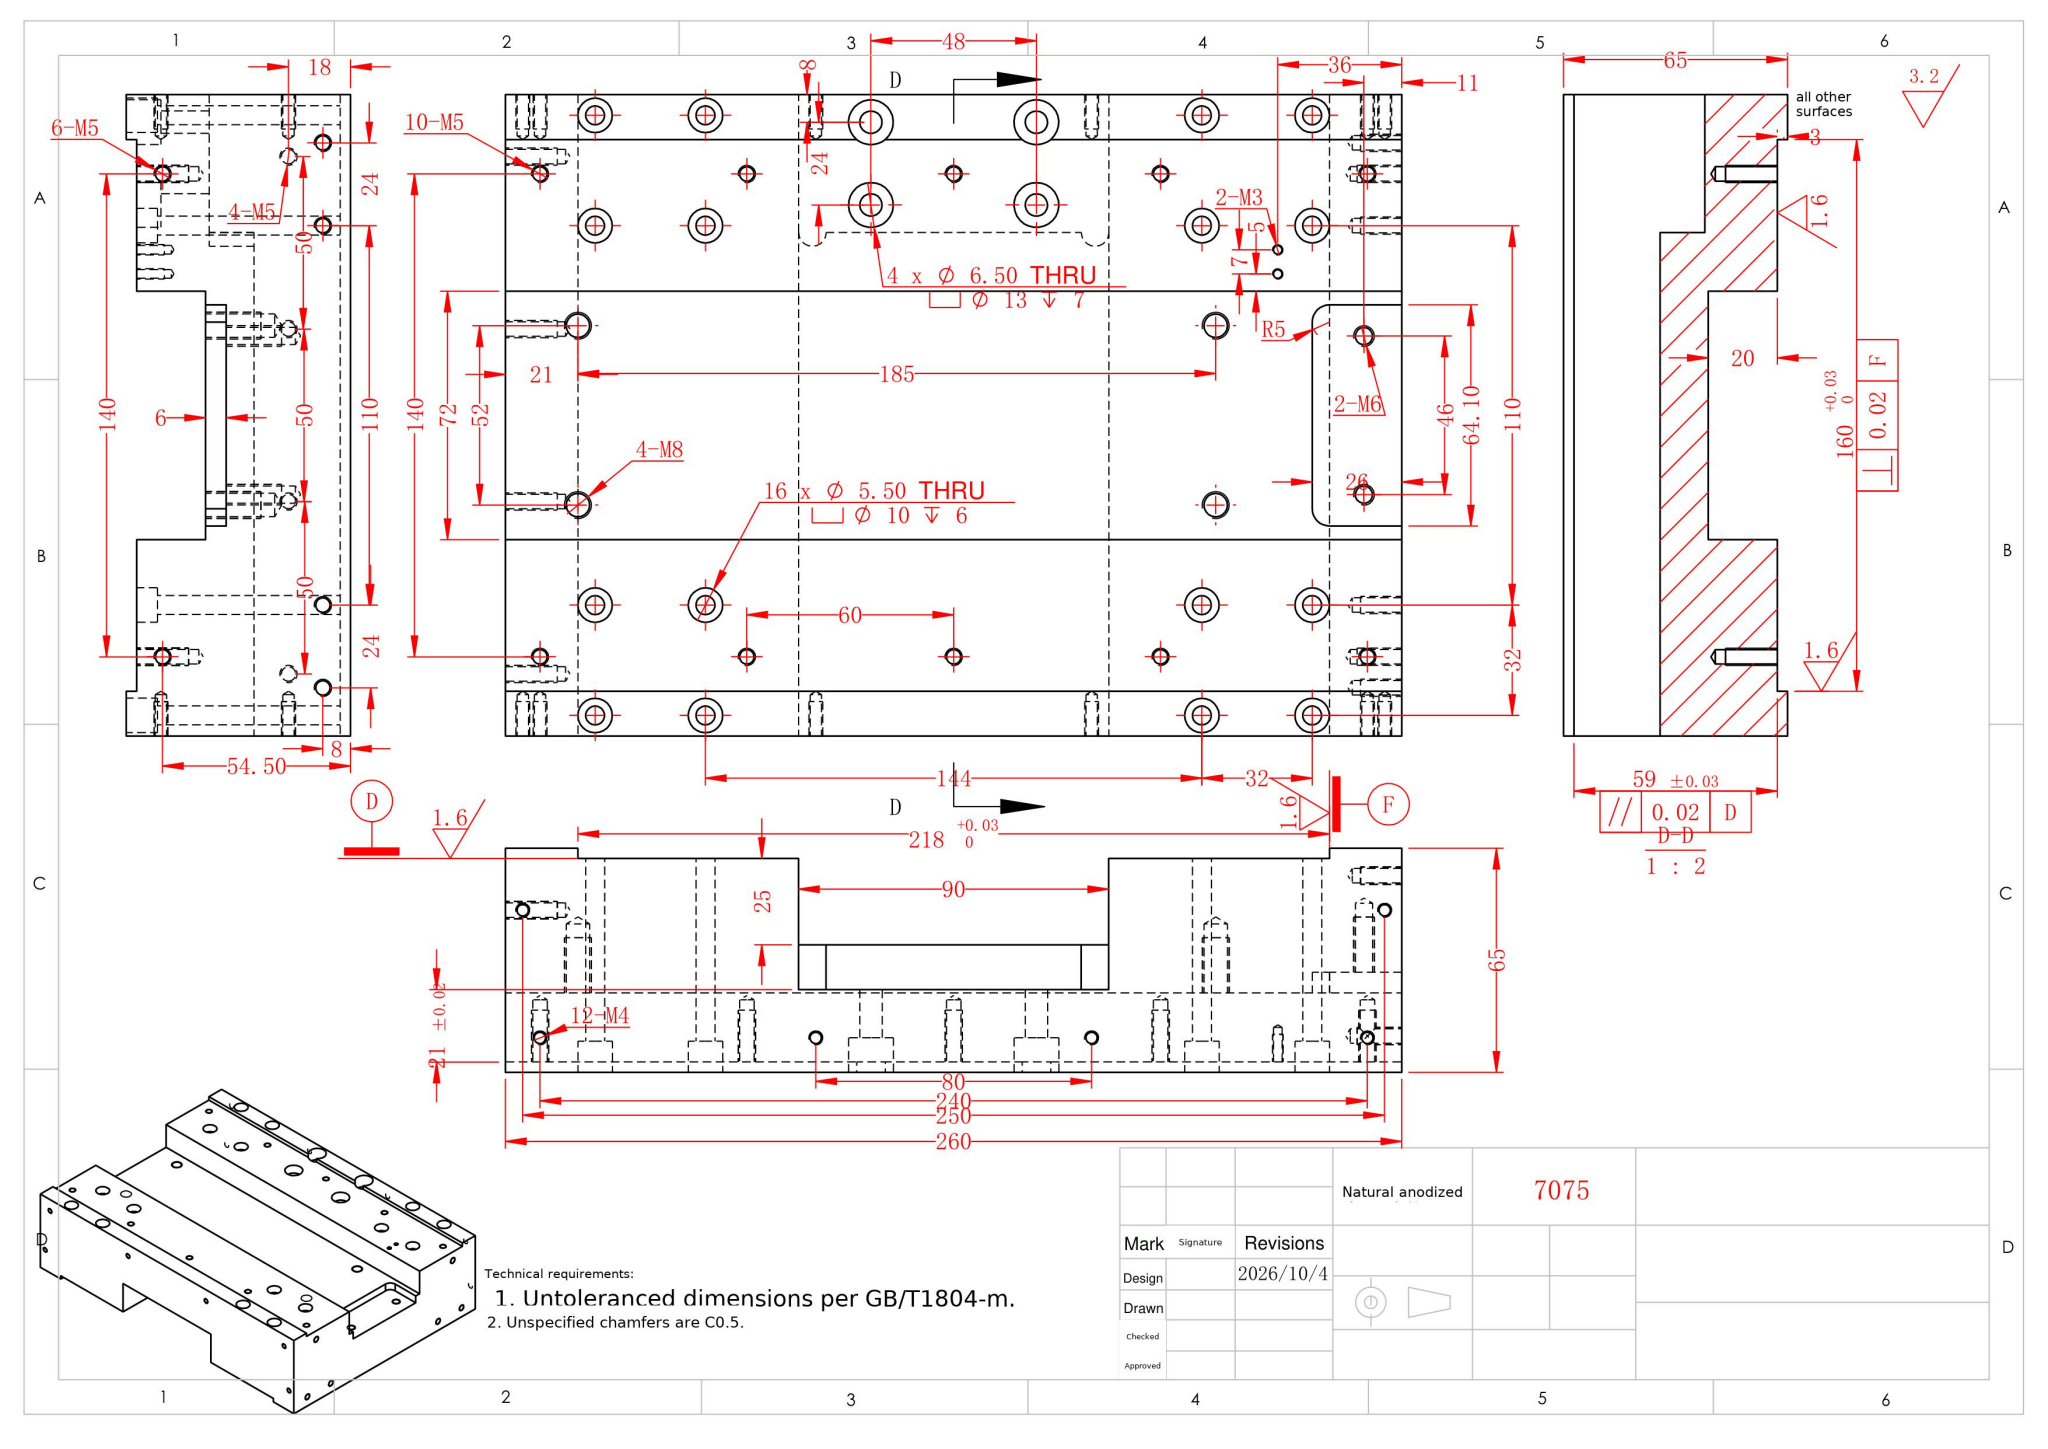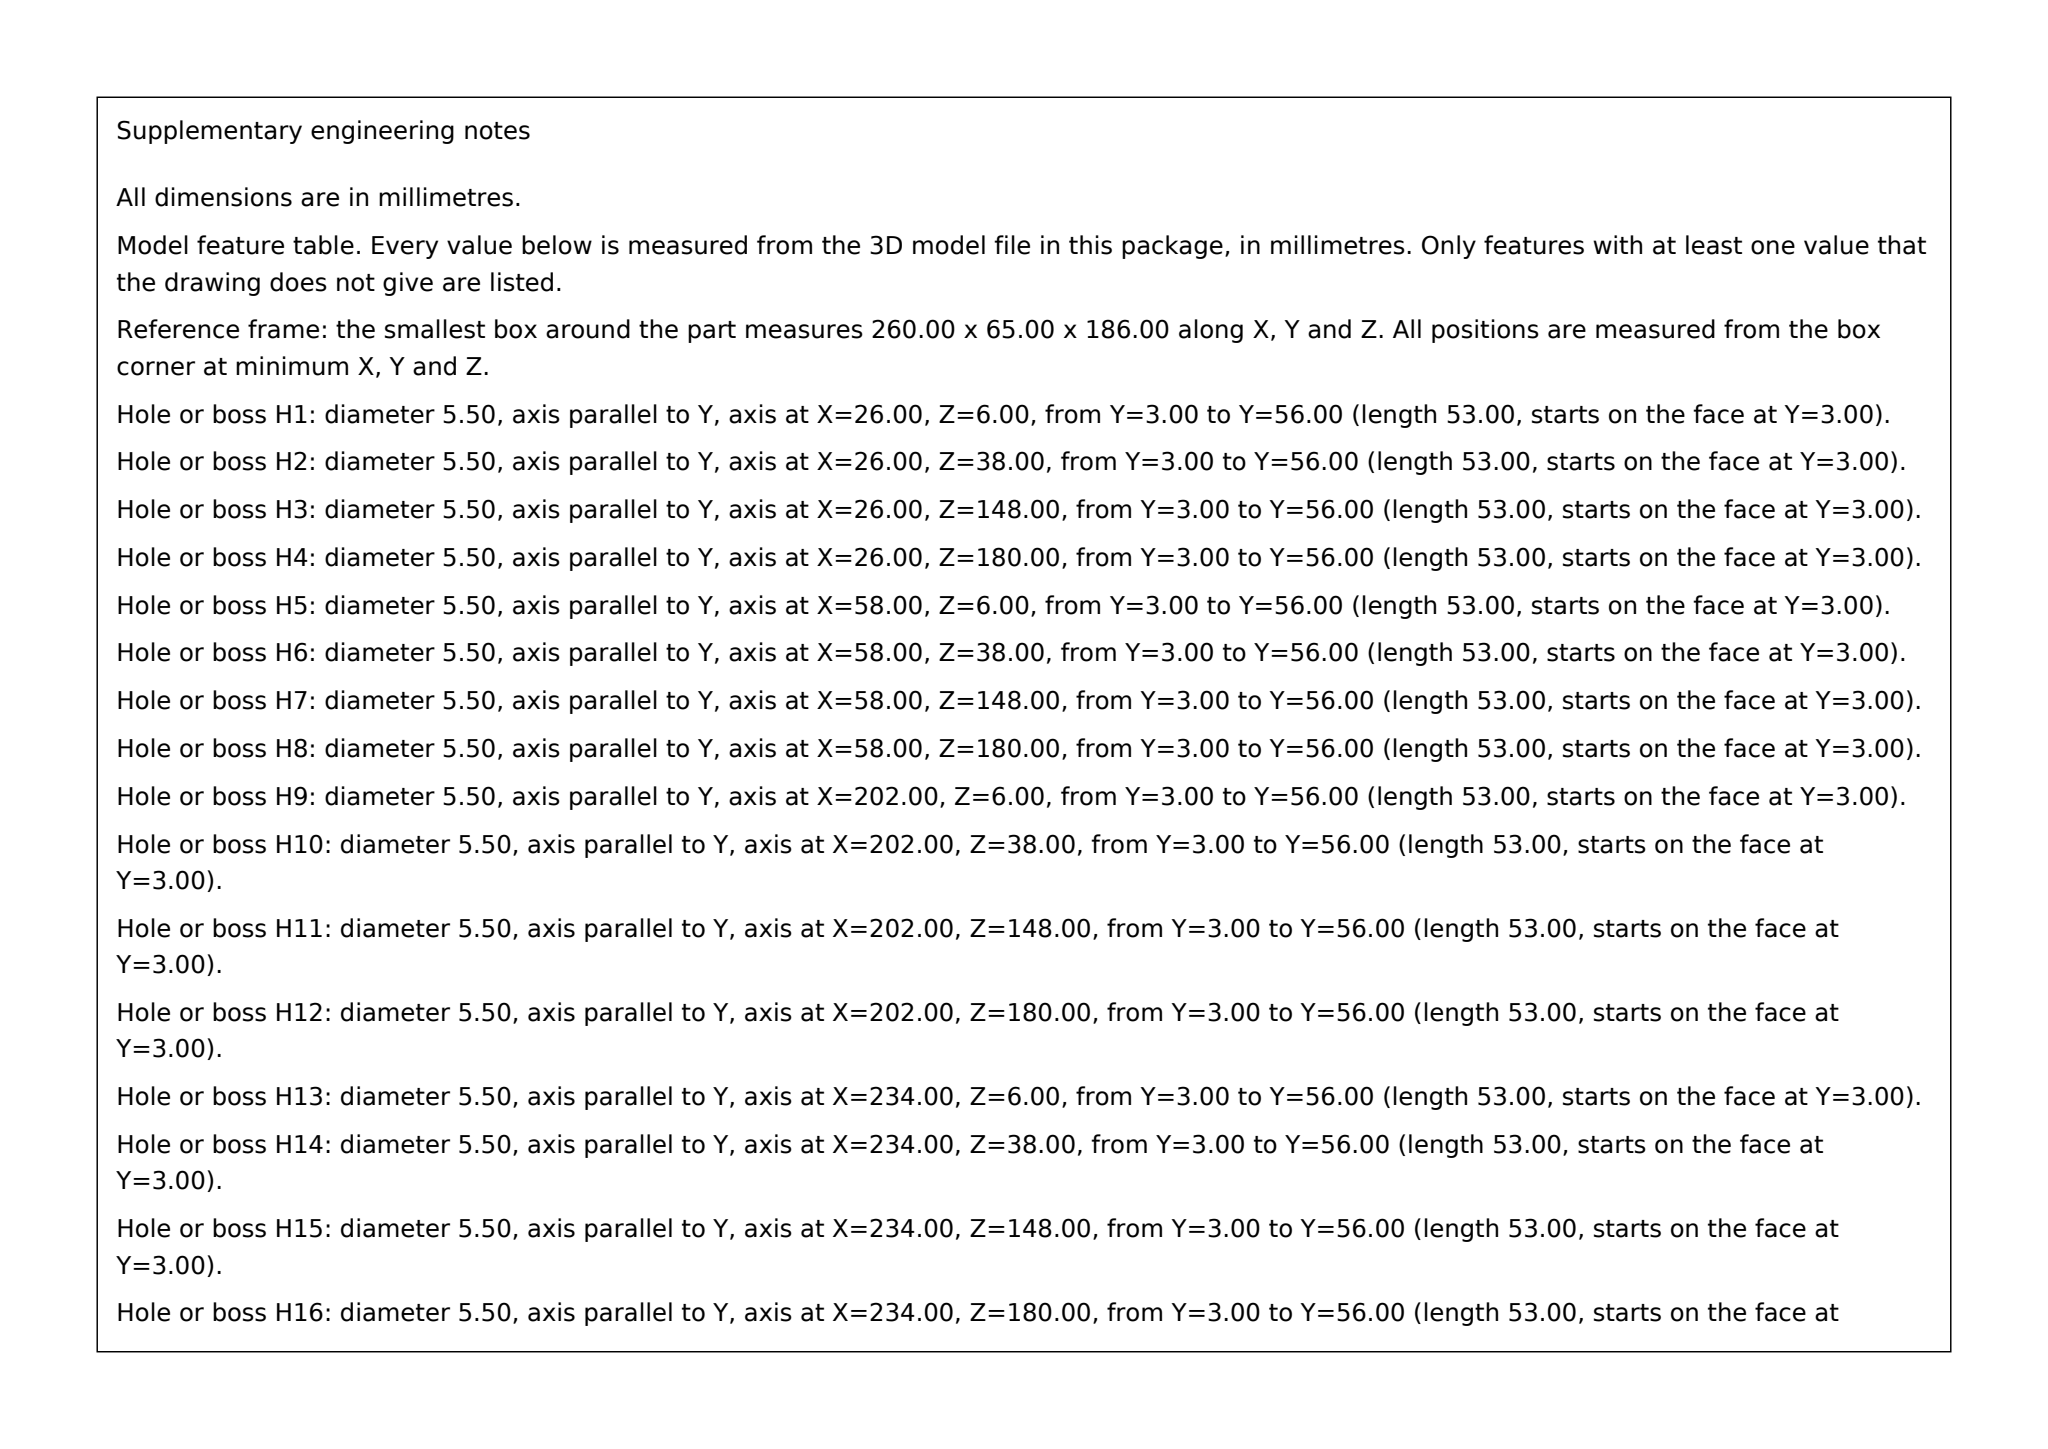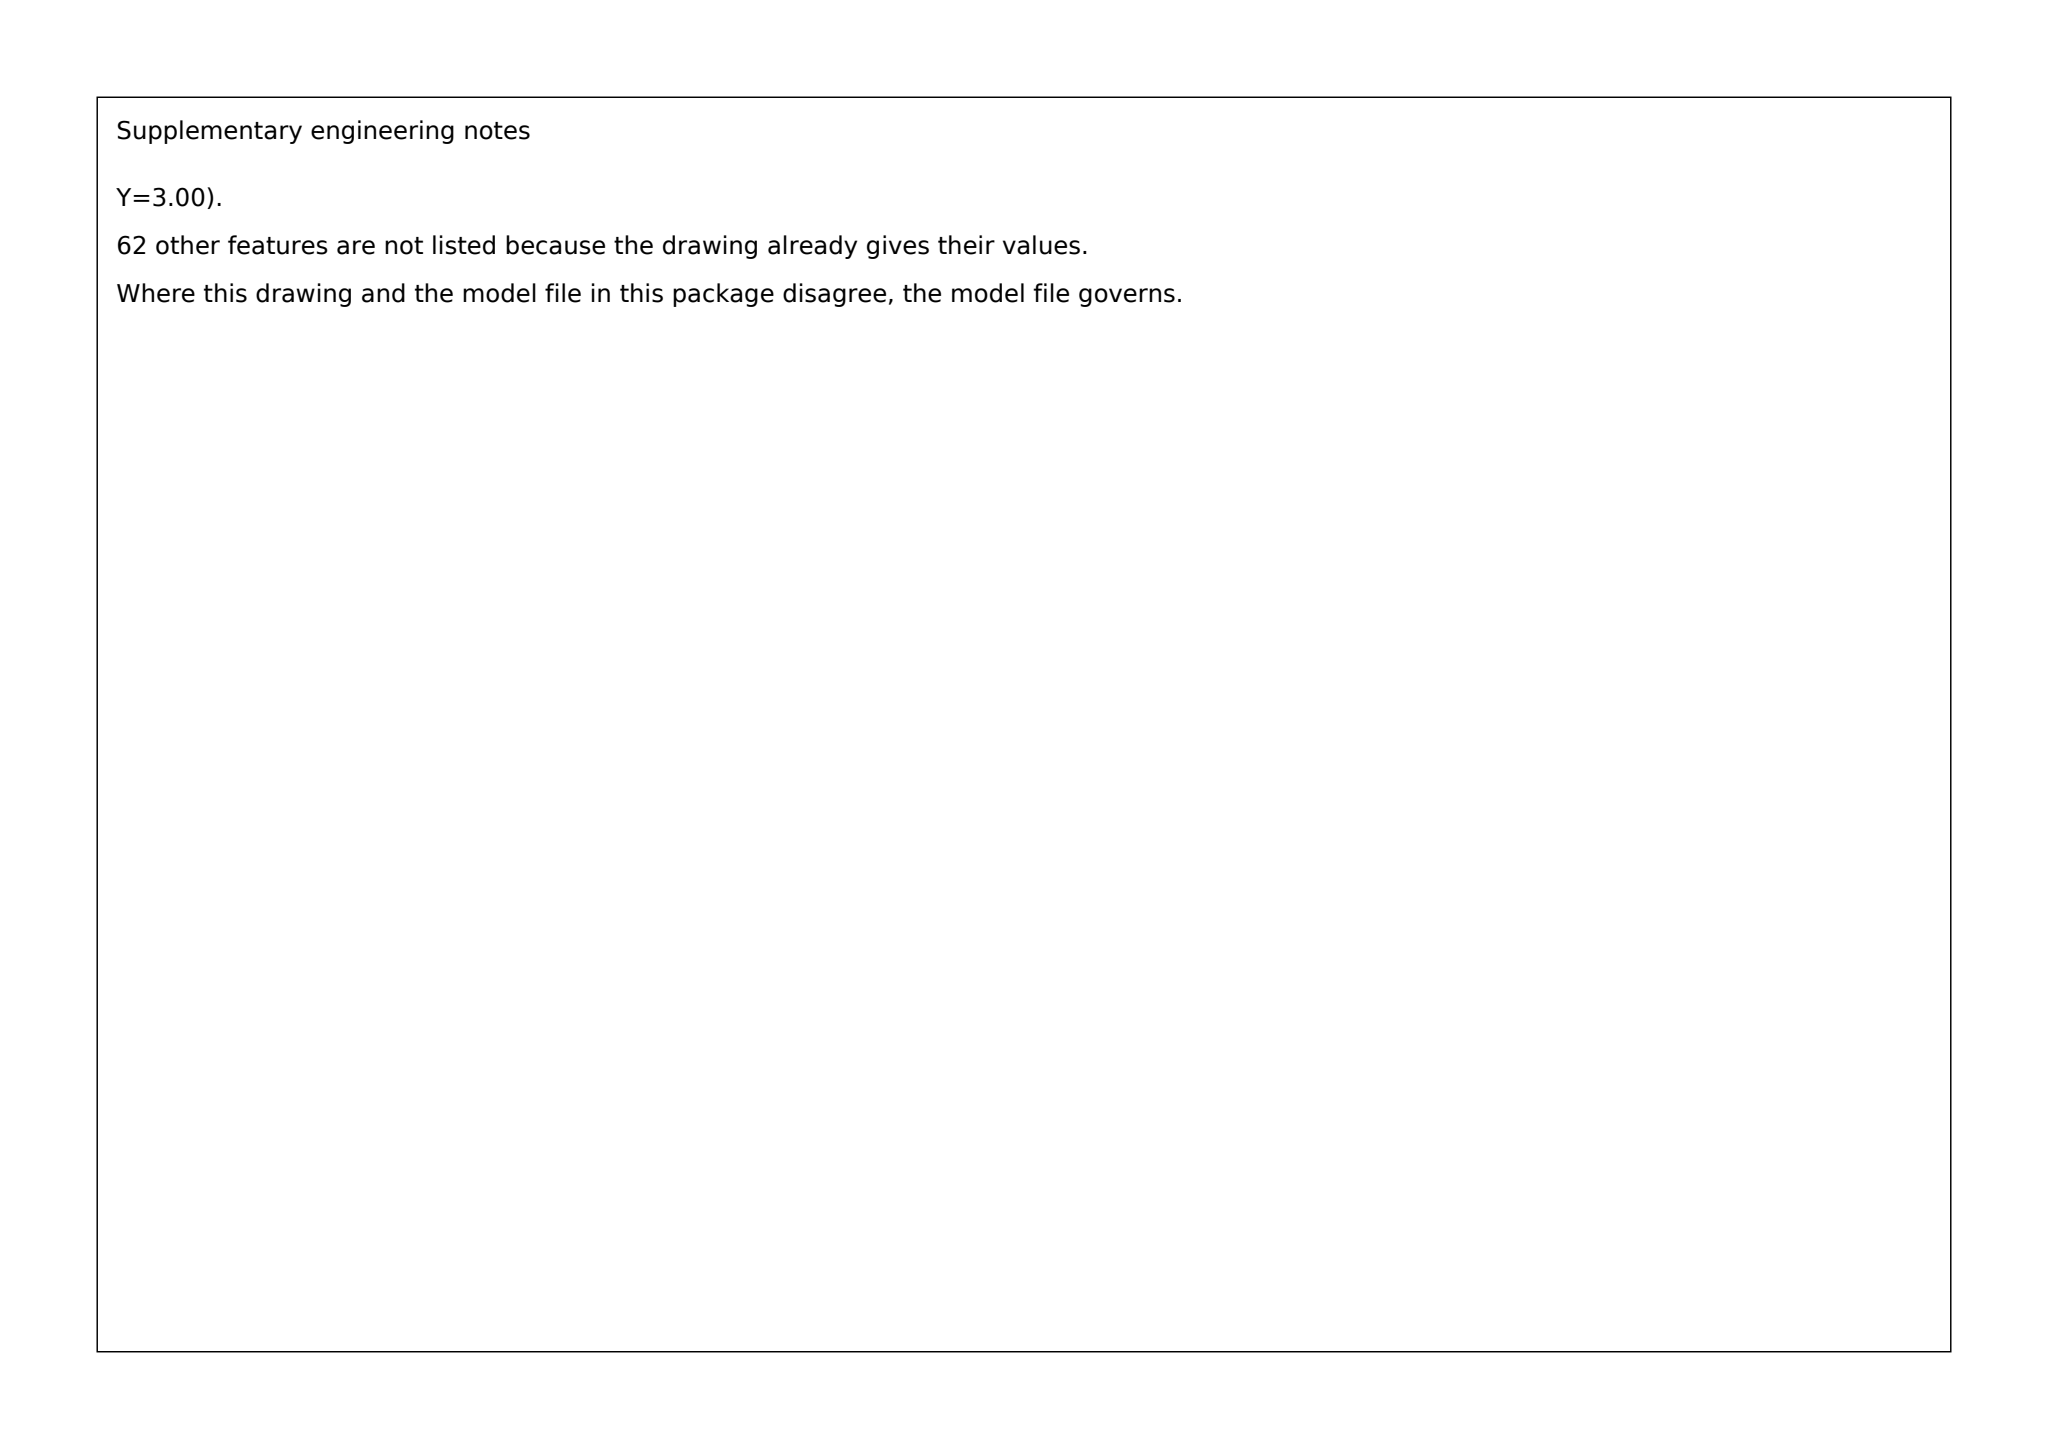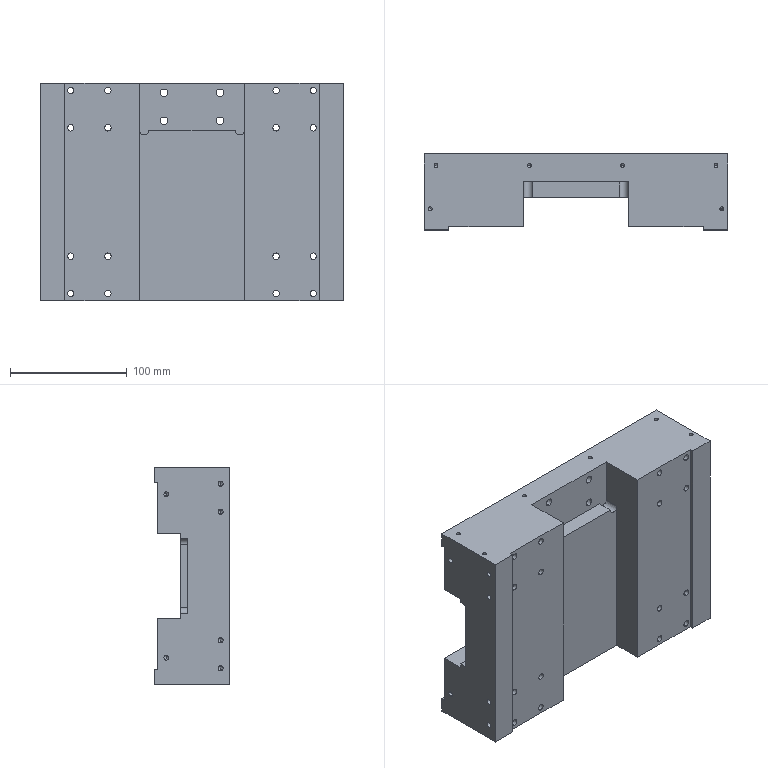Part | SolidWorks | mm | material 7075 | 1 solid | 302 faces | box 260 x 65 x 186 mm | volume 2000911 mm3 | cylinder 172 | cone 80 | plane 50 | commonest cylinder face diameters 4.2 x48 10 x34 5.5 x32 3.3 x24 6.8 x8 13 x8 6.5 x8 2.5 x4